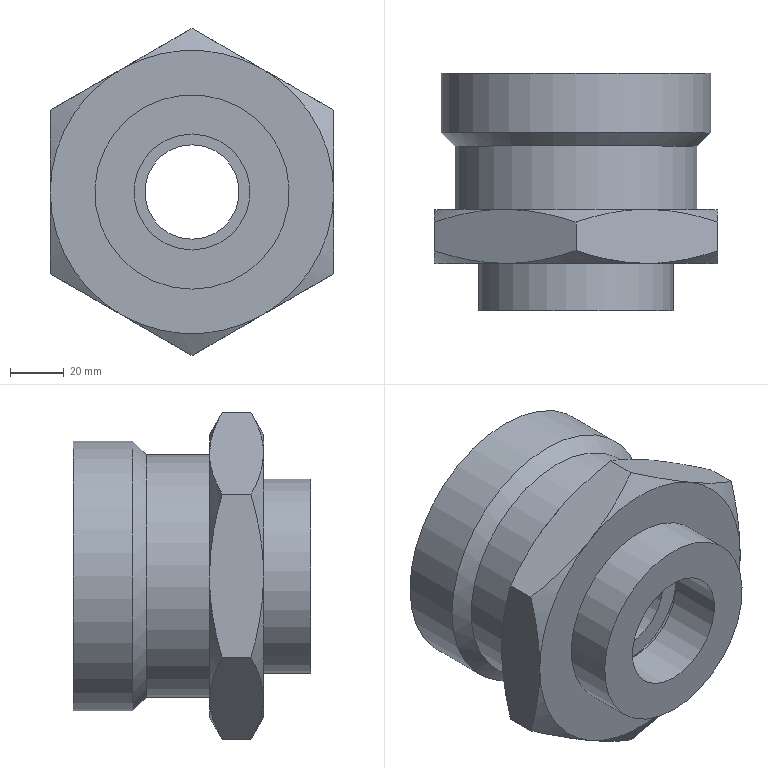Component | NX | HINGE_BODY | 1 solid | 35 faces | volume 315972 mm3 | plane 14 | cone 13 | cylinder 8 | commonest cylinder face diameters 90 x1 43 x1 49 x1 35 x1 82 x1 80 x1 100 x1 72 x1